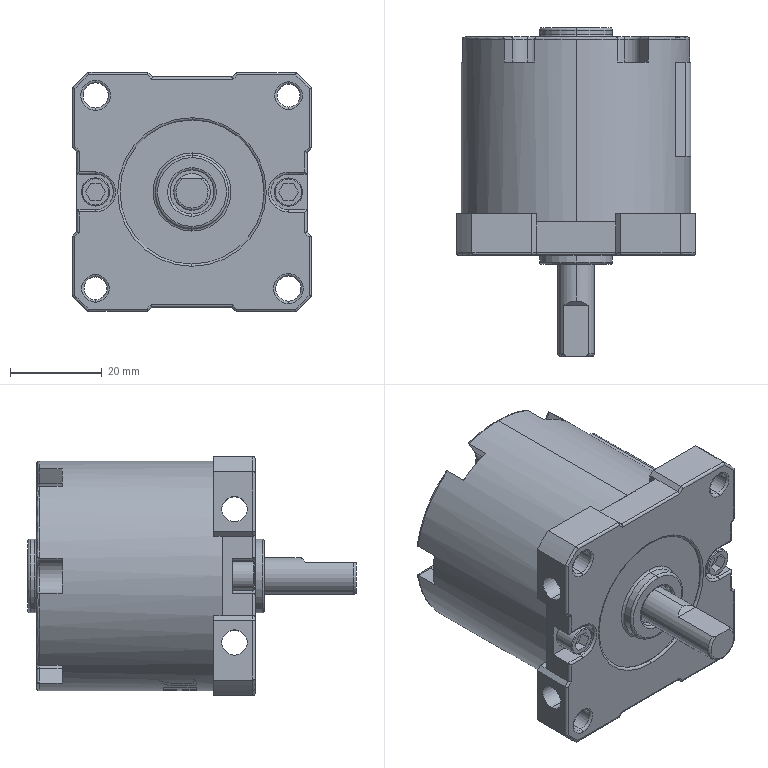Component | SolidWorks | VaneRotaryActuatorCRBU2S30-180-1 | 1 solid | 285 faces | box 52.05 x 71.5 x 52.05 mm | volume 94675 mm3 | plane 123 | cylinder 100 | torus 51 | spline 11 | commonest cylinder face diameters 1 x38 5 x18 7.7 x10 5.5 x8 6.16 x4 16 x4 49.98 x4 69 x4